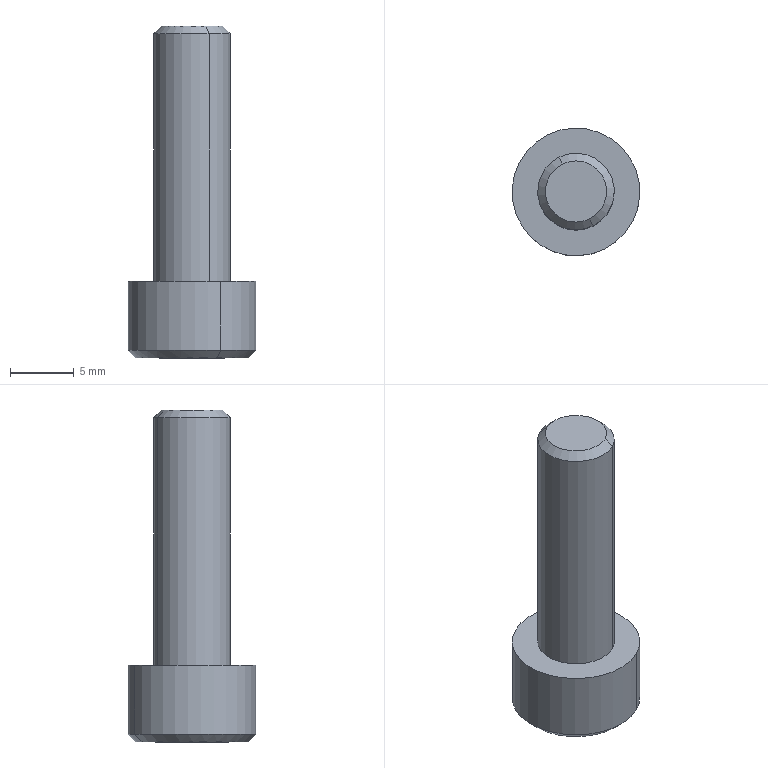Component | SolidWorks | LD101-02-HexagonScrew-M6-2-6 | 1 solid | 25 faces | box 10 x 10 x 26 mm | volume 959 mm3 | plane 15 | cone 6 | cylinder 4 | commonest cylinder face diameters 10 x2 6 x2
STEP:
#1=COLOUR_RGB('',0.7922,0.8196,0.9333);
#2=FILL_AREA_STYLE_COLOUR('',#1);
#3=FILL_AREA_STYLE('',(#2));
#4=SURFACE_STYLE_FILL_AREA(#3);
#5=SURFACE_SIDE_STYLE('',(#4));
#6=SURFACE_STYLE_USAGE(.BOTH.,#5);
#7=PRESENTATION_STYLE_ASSIGNMENT((#6));
#8=CARTESIAN_POINT('',(3.096,-6.841,0.2857));
#9=VERTEX_POINT('',#8);
#10=CARTESIAN_POINT('',(3.18,-7.01,0.2857));
#11=VERTEX_POINT('',#10);
#12=CARTESIAN_POINT('',(3.138,-6.925,0.2857));
#13=DIRECTION('',(0.,0.,1.));
#14=DIRECTION('',(-0.4466,0.8947,0.));
#15=AXIS2_PLACEMENT_3D('',#12,#13,#14);
#16=CIRCLE('',#15,0.09449);
#17=EDGE_CURVE('',#9,#11,#16,.T.);
#18=ORIENTED_EDGE('',*,*,#17,.F.);
#19=CARTESIAN_POINT('',(3.085,-6.819,0.2621));
#20=VERTEX_POINT('',#19);
#21=CARTESIAN_POINT('',(3.096,-6.841,0.2857));
#22=DIRECTION('',(-0.3158,0.6327,-0.7071));
#23=VECTOR('',#22,39.37);
#24=LINE('',#21,#23);
#25=EDGE_CURVE('',#9,#20,#24,.T.);
#26=ORIENTED_EDGE('',*,*,#25,.T.);
#27=CARTESIAN_POINT('',(3.191,-7.031,0.2621));
#28=VERTEX_POINT('',#27);
#29=CARTESIAN_POINT('',(3.138,-6.925,0.2621));
#30=DIRECTION('',(0.,0.,-1.));
#31=DIRECTION('',(-0.4466,0.8947,0.));
#32=AXIS2_PLACEMENT_3D('',#29,#30,#31);
#33=CIRCLE('',#32,0.1181);
#34=EDGE_CURVE('',#28,#20,#33,.T.);
#35=ORIENTED_EDGE('',*,*,#34,.F.);
#36=CARTESIAN_POINT('',(3.18,-7.01,0.2857));
#37=DIRECTION('',(0.3158,-0.6327,-0.7071));
#38=VECTOR('',#37,39.37);
#39=LINE('',#36,#38);
#40=EDGE_CURVE('',#11,#28,#39,.T.);
#41=ORIENTED_EDGE('',*,*,#40,.F.);
#42=EDGE_LOOP('',(#18,#26,#35,#41));
#43=FACE_OUTER_BOUND('',#42,.T.);
#44=CARTESIAN_POINT('',(3.138,-6.925,0.2857));
#45=DIRECTION('',(0.,0.,-1.));
#46=DIRECTION('',(0.4466,-0.8947,0.));
#47=AXIS2_PLACEMENT_3D('',#44,#45,#46);
#48=CONICAL_SURFACE('',#47,0.09449,0.7854);
#49=ADVANCED_FACE('',(#43),#48,.T.);
#50=CARTESIAN_POINT('',(3.05,-6.749,-0.7143));
#51=VERTEX_POINT('',#50);
#52=CARTESIAN_POINT('',(3.226,-7.101,-0.7143));
#53=VERTEX_POINT('',#52);
#54=CARTESIAN_POINT('',(3.138,-6.925,-0.7143));
#55=DIRECTION('',(0.,0.,1.));
#56=DIRECTION('',(-0.4466,0.8947,0.));
#57=AXIS2_PLACEMENT_3D('',#54,#55,#56);
#58=CIRCLE('',#57,0.1969);
#59=EDGE_CURVE('',#51,#53,#58,.T.);
#60=ORIENTED_EDGE('',*,*,#59,.T.);
#61=CARTESIAN_POINT('',(3.226,-7.101,-0.5017));
#62=VERTEX_POINT('',#61);
#63=CARTESIAN_POINT('',(3.226,-7.101,-0.608));
#64=DIRECTION('',(0.,0.,1.));
#65=VECTOR('',#64,39.37);
#66=LINE('',#63,#65);
#67=EDGE_CURVE('',#53,#62,#66,.T.);
#68=ORIENTED_EDGE('',*,*,#67,.T.);
#69=CARTESIAN_POINT('',(3.05,-6.749,-0.5017));
#70=VERTEX_POINT('',#69);
#71=CARTESIAN_POINT('',(3.138,-6.925,-0.5017));
#72=DIRECTION('',(0.,0.,-1.));
#73=DIRECTION('',(-0.4466,0.8947,0.));
#74=AXIS2_PLACEMENT_3D('',#71,#72,#73);
#75=CIRCLE('',#74,0.1969);
#76=EDGE_CURVE('',#62,#70,#75,.T.);
#77=ORIENTED_EDGE('',*,*,#76,.T.);
#78=CARTESIAN_POINT('',(3.05,-6.749,-0.608));
#79=DIRECTION('',(0.,0.,1.));
#80=VECTOR('',#79,39.37);
#81=LINE('',#78,#80);
#82=EDGE_CURVE('',#51,#70,#81,.T.);
#83=ORIENTED_EDGE('',*,*,#82,.F.);
#84=EDGE_LOOP('',(#60,#68,#77,#83));
#85=FACE_OUTER_BOUND('',#84,.T.);
#86=CARTESIAN_POINT('',(3.138,-6.925,-0.608));
#87=DIRECTION('',(0.,0.,1.));
#88=DIRECTION('',(-0.4466,0.8947,0.));
#89=AXIS2_PLACEMENT_3D('',#86,#87,#88);
#90=CYLINDRICAL_SURFACE('',#89,0.1969);
#91=ADVANCED_FACE('',(#85),#90,.T.);
#92=CARTESIAN_POINT('',(3.061,-6.77,-0.7379));
#93=VERTEX_POINT('',#92);
#94=CARTESIAN_POINT('',(3.216,-7.08,-0.7379));
#95=VERTEX_POINT('',#94);
#96=CARTESIAN_POINT('',(3.138,-6.925,-0.7379));
#97=DIRECTION('',(0.,0.,1.));
#98=DIRECTION('',(-0.4466,0.8947,0.));
#99=AXIS2_PLACEMENT_3D('',#96,#97,#98);
#100=CIRCLE('',#99,0.1732);
#101=EDGE_CURVE('',#93,#95,#100,.T.);
#102=ORIENTED_EDGE('',*,*,#101,.T.);
#103=CARTESIAN_POINT('',(3.226,-7.101,-0.7143));
#104=DIRECTION('',(0.3158,-0.6327,0.7071));
#105=VECTOR('',#104,39.37);
#106=LINE('',#103,#105);
#107=EDGE_CURVE('',#95,#53,#106,.T.);
#108=ORIENTED_EDGE('',*,*,#107,.T.);
#109=ORIENTED_EDGE('',*,*,#59,.F.);
#110=CARTESIAN_POINT('',(3.05,-6.749,-0.7143));
#111=DIRECTION('',(-0.3158,0.6327,0.7071));
#112=VECTOR('',#111,39.37);
#113=LINE('',#110,#112);
#114=EDGE_CURVE('',#93,#51,#113,.T.);
#115=ORIENTED_EDGE('',*,*,#114,.F.);
#116=EDGE_LOOP('',(#102,#108,#109,#115));
#117=FACE_OUTER_BOUND('',#116,.T.);
#118=CARTESIAN_POINT('',(3.138,-6.925,-0.7143));
#119=DIRECTION('',(0.,0.,1.));
#120=DIRECTION('',(-0.4466,0.8947,0.));
#121=AXIS2_PLACEMENT_3D('',#118,#119,#120);
#122=CONICAL_SURFACE('',#121,0.1969,0.7854);
#123=ADVANCED_FACE('',(#117),#122,.T.);
#124=CARTESIAN_POINT('',(3.191,-7.031,-0.5017));
#125=VERTEX_POINT('',#124);
#126=CARTESIAN_POINT('',(3.085,-6.819,-0.5017));
#127=VERTEX_POINT('',#126);
#128=CARTESIAN_POINT('',(3.138,-6.925,-0.5017));
#129=DIRECTION('',(0.,0.,-1.));
#130=DIRECTION('',(-0.4466,0.8947,0.));
#131=AXIS2_PLACEMENT_3D('',#128,#129,#130);
#132=CIRCLE('',#131,0.1181);
#133=EDGE_CURVE('',#125,#127,#132,.T.);
#134=ORIENTED_EDGE('',*,*,#133,.F.);
#135=CARTESIAN_POINT('',(3.191,-7.031,-0.3563));
#136=DIRECTION('',(0.,0.,1.));
#137=VECTOR('',#136,39.37);
#138=LINE('',#135,#137);
#139=EDGE_CURVE('',#125,#28,#138,.T.);
#140=ORIENTED_EDGE('',*,*,#139,.T.);
#141=ORIENTED_EDGE('',*,*,#34,.T.);
#142=CARTESIAN_POINT('',(3.085,-6.819,-0.3563));
#143=DIRECTION('',(0.,0.,1.));
#144=VECTOR('',#143,39.37);
#145=LINE('',#142,#144);
#146=EDGE_CURVE('',#127,#20,#145,.T.);
#147=ORIENTED_EDGE('',*,*,#146,.F.);
#148=EDGE_LOOP('',(#134,#140,#141,#147));
#149=FACE_OUTER_BOUND('',#148,.T.);
#150=CARTESIAN_POINT('',(3.138,-6.925,-0.3563));
#151=DIRECTION('',(0.,0.,1.));
#152=DIRECTION('',(-0.4466,0.8947,0.));
#153=AXIS2_PLACEMENT_3D('',#150,#151,#152);
#154=CYLINDRICAL_SURFACE('',#153,0.1181);
#155=ADVANCED_FACE('',(#149),#154,.T.);
#156=CARTESIAN_POINT('',(3.138,-6.925,-0.5934));
#157=VERTEX_POINT('',#156);
#158=CARTESIAN_POINT('',(3.182,-7.013,-0.6198));
#159=VERTEX_POINT('',#158);
#160=CARTESIAN_POINT('',(3.182,-7.013,-0.6198));
#161=DIRECTION('',(0.4314,-0.8642,-0.2588));
#162=VECTOR('',#161,39.37);
#163=LINE('',#160,#162);
#164=EDGE_CURVE('',#157,#159,#163,.T.);
#165=ORIENTED_EDGE('',*,*,#164,.F.);
#166=CARTESIAN_POINT('',(3.094,-6.837,-0.6198));
#167=VERTEX_POINT('',#166);
#168=CARTESIAN_POINT('',(3.094,-6.837,-0.6198));
#169=DIRECTION('',(-0.4314,0.8642,-0.2588));
#170=VECTOR('',#169,39.37);
#171=LINE('',#168,#170);
#172=EDGE_CURVE('',#157,#167,#171,.T.);
#173=ORIENTED_EDGE('',*,*,#172,.T.);
#174=CARTESIAN_POINT('',(3.192,-6.843,-0.6198));
#175=VERTEX_POINT('',#174);
#176=CARTESIAN_POINT('',(3.138,-6.925,-0.6198));
#177=DIRECTION('',(0.,-0.,1.));
#178=DIRECTION('',(0.4466,-0.8947,0.));
#179=AXIS2_PLACEMENT_3D('',#176,#177,#178);
#180=CIRCLE('',#179,0.09843);
#181=EDGE_CURVE('',#175,#167,#180,.T.);
#182=ORIENTED_EDGE('',*,*,#181,.F.);
#183=CARTESIAN_POINT('',(3.236,-6.931,-0.6198));
#184=VERTEX_POINT('',#183);
#185=CARTESIAN_POINT('',(3.138,-6.925,-0.6198));
#186=DIRECTION('',(0.,-0.,1.));
#187=DIRECTION('',(0.4466,-0.8947,0.));
#188=AXIS2_PLACEMENT_3D('',#185,#186,#187);
#189=CIRCLE('',#188,0.09843);
#190=EDGE_CURVE('',#184,#175,#189,.T.);
#191=ORIENTED_EDGE('',*,*,#190,.F.);
#192=CARTESIAN_POINT('',(3.138,-6.925,-0.6198));
#193=DIRECTION('',(-0.,0.,-1.));
#194=DIRECTION('',(0.4466,-0.8947,0.));
#195=AXIS2_PLACEMENT_3D('',#192,#193,#194);
#196=CIRCLE('',#195,0.09843);
#197=EDGE_CURVE('',#184,#159,#196,.T.);
#198=ORIENTED_EDGE('',*,*,#197,.T.);
#199=EDGE_LOOP('',(#165,#173,#182,#191,#198));
#200=FACE_OUTER_BOUND('',#199,.T.);
#201=CARTESIAN_POINT('',(3.138,-6.925,-0.6198));
#202=DIRECTION('',(-0.,0.,-1.));
#203=DIRECTION('',(0.4466,-0.8947,0.));
#204=AXIS2_PLACEMENT_3D('',#201,#202,#203);
#205=CONICAL_SURFACE('',#204,0.09843,1.309);
#206=ADVANCED_FACE('',(#200),#205,.F.);
#207=ORIENTED_EDGE('',*,*,#67,.F.);
#208=CARTESIAN_POINT('',(3.138,-6.925,-0.7143));
#209=DIRECTION('',(0.,0.,1.));
#210=DIRECTION('',(-0.4466,0.8947,0.));
#211=AXIS2_PLACEMENT_3D('',#208,#209,#210);
#212=CIRCLE('',#211,0.1969);
#213=EDGE_CURVE('',#53,#51,#212,.T.);
#214=ORIENTED_EDGE('',*,*,#213,.T.);
#215=ORIENTED_EDGE('',*,*,#82,.T.);
#216=CARTESIAN_POINT('',(3.138,-6.925,-0.5017));
#217=DIRECTION('',(0.,0.,-1.));
#218=DIRECTION('',(-0.4466,0.8947,0.));
#219=AXIS2_PLACEMENT_3D('',#216,#217,#218);
#220=CIRCLE('',#219,0.1969);
#221=EDGE_CURVE('',#70,#62,#220,.T.);
#222=ORIENTED_EDGE('',*,*,#221,.T.);
#223=EDGE_LOOP('',(#207,#214,#215,#222));
#224=FACE_OUTER_BOUND('',#223,.T.);
#225=CARTESIAN_POINT('',(3.138,-6.925,-0.608));
#226=DIRECTION('',(0.,0.,1.));
#227=DIRECTION('',(-0.4466,0.8947,0.));
#228=AXIS2_PLACEMENT_3D('',#225,#226,#227);
#229=CYLINDRICAL_SURFACE('',#228,0.1969);
#230=ADVANCED_FACE('',(#224),#229,.T.);
#231=ORIENTED_EDGE('',*,*,#107,.F.);
#232=CARTESIAN_POINT('',(3.138,-6.925,-0.7379));
#233=DIRECTION('',(0.,0.,1.));
#234=DIRECTION('',(-0.4466,0.8947,0.));
#235=AXIS2_PLACEMENT_3D('',#232,#233,#234);
#236=CIRCLE('',#235,0.1732);
#237=EDGE_CURVE('',#95,#93,#236,.T.);
#238=ORIENTED_EDGE('',*,*,#237,.T.);
#239=ORIENTED_EDGE('',*,*,#114,.T.);
#240=ORIENTED_EDGE('',*,*,#213,.F.);
#241=EDGE_LOOP('',(#231,#238,#239,#240));
#242=FACE_OUTER_BOUND('',#241,.T.);
#243=CARTESIAN_POINT('',(3.138,-6.925,-0.7143));
#244=DIRECTION('',(0.,0.,1.));
#245=DIRECTION('',(-0.4466,0.8947,0.));
#246=AXIS2_PLACEMENT_3D('',#243,#244,#245);
#247=CONICAL_SURFACE('',#246,0.1969,0.7854);
#248=ADVANCED_FACE('',(#242),#247,.T.);
#249=CARTESIAN_POINT('',(3.138,-6.925,-0.5017));
#250=DIRECTION('',(0.,0.,-1.));
#251=DIRECTION('',(-0.4466,0.8947,0.));
#252=AXIS2_PLACEMENT_3D('',#249,#250,#251);
#253=CIRCLE('',#252,0.1181);
#254=EDGE_CURVE('',#127,#125,#253,.T.);
#255=ORIENTED_EDGE('',*,*,#254,.T.);
#256=ORIENTED_EDGE('',*,*,#133,.T.);
#257=EDGE_LOOP('',(#255,#256));
#258=FACE_BOUND('',#257,.T.);
#259=ORIENTED_EDGE('',*,*,#221,.F.);
#260=ORIENTED_EDGE('',*,*,#76,.F.);
#261=EDGE_LOOP('',(#259,#260));
#262=FACE_OUTER_BOUND('',#261,.T.);
#263=CARTESIAN_POINT('',(2.997,-6.995,-0.5017));
#264=DIRECTION('',(0.,0.,1.));
#265=DIRECTION('',(-0.4466,0.8947,0.));
#266=AXIS2_PLACEMENT_3D('',#263,#264,#265);
#267=PLANE('',#266);
#268=ADVANCED_FACE('',(#258,#262),#267,.T.);
#269=ORIENTED_EDGE('',*,*,#101,.F.);
#270=ORIENTED_EDGE('',*,*,#237,.F.);
#271=EDGE_LOOP('',(#269,#270));
#272=FACE_OUTER_BOUND('',#271,.T.);
#273=CARTESIAN_POINT('',(3.043,-6.862,-0.7379));
#274=VERTEX_POINT('',#273);
#275=CARTESIAN_POINT('',(3.037,-6.976,-0.7379));
#276=VERTEX_POINT('',#275);
#277=CARTESIAN_POINT('',(3.043,-6.862,-0.7379));
#278=DIRECTION('',(-0.06055,-0.9982,0.));
#279=VECTOR('',#278,39.37);
#280=LINE('',#277,#279);
#281=EDGE_CURVE('',#274,#276,#280,.T.);
#282=ORIENTED_EDGE('',*,*,#281,.T.);
#283=CARTESIAN_POINT('',(3.131,-7.039,-0.7379));
#284=VERTEX_POINT('',#283);
#285=CARTESIAN_POINT('',(3.037,-6.976,-0.7379));
#286=DIRECTION('',(0.8342,-0.5515,0.));
#287=VECTOR('',#286,39.37);
#288=LINE('',#285,#287);
#289=EDGE_CURVE('',#276,#284,#288,.T.);
#290=ORIENTED_EDGE('',*,*,#289,.T.);
#291=CARTESIAN_POINT('',(3.233,-6.988,-0.7379));
#292=VERTEX_POINT('',#291);
#293=CARTESIAN_POINT('',(3.105,-7.052,-0.7379));
#294=DIRECTION('',(0.8947,0.4466,0.));
#295=VECTOR('',#294,39.37);
#296=LINE('',#293,#295);
#297=EDGE_CURVE('',#284,#292,#296,.T.);
#298=ORIENTED_EDGE('',*,*,#297,.T.);
#299=CARTESIAN_POINT('',(3.24,-6.874,-0.7379));
#300=VERTEX_POINT('',#299);
#301=CARTESIAN_POINT('',(3.233,-6.988,-0.7379));
#302=DIRECTION('',(0.06055,0.9982,0.));
#303=VECTOR('',#302,39.37);
#304=LINE('',#301,#303);
#305=EDGE_CURVE('',#292,#300,#304,.T.);
#306=ORIENTED_EDGE('',*,*,#305,.T.);
#307=CARTESIAN_POINT('',(3.145,-6.812,-0.7379));
#308=VERTEX_POINT('',#307);
#309=CARTESIAN_POINT('',(3.24,-6.874,-0.7379));
#310=DIRECTION('',(-0.8342,0.5515,0.));
#311=VECTOR('',#310,39.37);
#312=LINE('',#309,#311);
#313=EDGE_CURVE('',#300,#308,#312,.T.);
#314=ORIENTED_EDGE('',*,*,#313,.T.);
#315=CARTESIAN_POINT('',(3.017,-6.876,-0.7379));
#316=DIRECTION('',(-0.8947,-0.4466,0.));
#317=VECTOR('',#316,39.37);
#318=LINE('',#315,#317);
#319=EDGE_CURVE('',#308,#274,#318,.T.);
#320=ORIENTED_EDGE('',*,*,#319,.T.);
#321=EDGE_LOOP('',(#282,#290,#298,#306,#314,#320));
#322=FACE_BOUND('',#321,.T.);
#323=CARTESIAN_POINT('',(3.061,-6.964,-0.7379));
#324=DIRECTION('',(0.,0.,-1.));
#325=DIRECTION('',(0.4466,-0.8947,0.));
#326=AXIS2_PLACEMENT_3D('',#323,#324,#325);
#327=PLANE('',#326);
#328=ADVANCED_FACE('',(#272,#322),#327,.T.);
#329=ORIENTED_EDGE('',*,*,#139,.F.);
#330=ORIENTED_EDGE('',*,*,#254,.F.);
#331=ORIENTED_EDGE('',*,*,#146,.T.);
#332=CARTESIAN_POINT('',(3.138,-6.925,0.2621));
#333=DIRECTION('',(0.,0.,-1.));
#334=DIRECTION('',(-0.4466,0.8947,0.));
#335=AXIS2_PLACEMENT_3D('',#332,#333,#334);
#336=CIRCLE('',#335,0.1181);
#337=EDGE_CURVE('',#20,#28,#336,.T.);
#338=ORIENTED_EDGE('',*,*,#337,.T.);
#339=EDGE_LOOP('',(#329,#330,#331,#338));
#340=FACE_OUTER_BOUND('',#339,.T.);
#341=CARTESIAN_POINT('',(3.138,-6.925,-0.3563));
#342=DIRECTION('',(0.,0.,1.));
#343=DIRECTION('',(-0.4466,0.8947,0.));
#344=AXIS2_PLACEMENT_3D('',#341,#342,#343);
#345=CYLINDRICAL_SURFACE('',#344,0.1181);
#346=ADVANCED_FACE('',(#340),#345,.T.);
#347=CARTESIAN_POINT('',(3.037,-6.976,-0.6198));
#348=VERTEX_POINT('',#347);
#349=CARTESIAN_POINT('',(3.037,-6.976,-0.7379));
#350=DIRECTION('',(0.,0.,-1.));
#351=VECTOR('',#350,39.37);
#352=LINE('',#349,#351);
#353=EDGE_CURVE('',#348,#276,#352,.T.);
#354=ORIENTED_EDGE('',*,*,#353,.F.);
#355=CARTESIAN_POINT('',(3.084,-7.007,-0.6198));
#356=VERTEX_POINT('',#355);
#357=CARTESIAN_POINT('',(3.131,-7.039,-0.6198));
#358=DIRECTION('',(-0.8342,0.5515,0.));
#359=VECTOR('',#358,39.37);
#360=LINE('',#357,#359);
#361=EDGE_CURVE('',#356,#348,#360,.T.);
#362=ORIENTED_EDGE('',*,*,#361,.F.);
#363=CARTESIAN_POINT('',(3.131,-7.039,-0.6198));
#364=VERTEX_POINT('',#363);
#365=CARTESIAN_POINT('',(3.084,-7.007,-0.6198));
#366=DIRECTION('',(0.8342,-0.5515,0.));
#367=VECTOR('',#366,39.37);
#368=LINE('',#365,#367);
#369=EDGE_CURVE('',#356,#364,#368,.T.);
#370=ORIENTED_EDGE('',*,*,#369,.T.);
#371=CARTESIAN_POINT('',(3.131,-7.039,-0.7379));
#372=DIRECTION('',(0.,0.,1.));
#373=VECTOR('',#372,39.37);
#374=LINE('',#371,#373);
#375=EDGE_CURVE('',#284,#364,#374,.T.);
#376=ORIENTED_EDGE('',*,*,#375,.F.);
#377=ORIENTED_EDGE('',*,*,#289,.F.);
#378=EDGE_LOOP('',(#354,#362,#370,#376,#377));
#379=FACE_OUTER_BOUND('',#378,.T.);
#380=CARTESIAN_POINT('',(3.131,-7.039,-0.7379));
#381=DIRECTION('',(-0.5515,-0.8342,0.));
#382=DIRECTION('',(0.8342,-0.5515,0.));
#383=AXIS2_PLACEMENT_3D('',#380,#381,#382);
#384=PLANE('',#383);
#385=ADVANCED_FACE('',(#379),#384,.F.);
#386=CARTESIAN_POINT('',(3.043,-6.862,-0.6198));
#387=VERTEX_POINT('',#386);
#388=CARTESIAN_POINT('',(3.043,-6.862,-0.7379));
#389=DIRECTION('',(0.,0.,-1.));
#390=VECTOR('',#389,39.37);
#391=LINE('',#388,#390);
#392=EDGE_CURVE('',#387,#274,#391,.T.);
#393=ORIENTED_EDGE('',*,*,#392,.F.);
#394=CARTESIAN_POINT('',(3.04,-6.919,-0.6198));
#395=VERTEX_POINT('',#394);
#396=CARTESIAN_POINT('',(3.043,-6.862,-0.6198));
#397=DIRECTION('',(-0.06055,-0.9982,0.));
#398=VECTOR('',#397,39.37);
#399=LINE('',#396,#398);
#400=EDGE_CURVE('',#387,#395,#399,.T.);
#401=ORIENTED_EDGE('',*,*,#400,.T.);
#402=CARTESIAN_POINT('',(3.037,-6.976,-0.6198));
#403=DIRECTION('',(0.06055,0.9982,0.));
#404=VECTOR('',#403,39.37);
#405=LINE('',#402,#404);
#406=EDGE_CURVE('',#348,#395,#405,.T.);
#407=ORIENTED_EDGE('',*,*,#406,.F.);
#408=ORIENTED_EDGE('',*,*,#353,.T.);
#409=ORIENTED_EDGE('',*,*,#281,.F.);
#410=EDGE_LOOP('',(#393,#401,#407,#408,#409));
#411=FACE_OUTER_BOUND('',#410,.T.);
#412=CARTESIAN_POINT('',(3.037,-6.976,-0.7379));
#413=DIRECTION('',(-0.9982,0.06055,0.));
#414=DIRECTION('',(-0.06055,-0.9982,0.));
#415=AXIS2_PLACEMENT_3D('',#412,#413,#414);
#416=PLANE('',#415);
#417=ADVANCED_FACE('',(#411),#416,.F.);
#418=CARTESIAN_POINT('',(3.145,-6.812,-0.6198));
#419=VERTEX_POINT('',#418);
#420=CARTESIAN_POINT('',(3.145,-6.812,-0.7379));
#421=DIRECTION('',(0.,0.,-1.));
#422=VECTOR('',#421,39.37);
#423=LINE('',#420,#422);
#424=EDGE_CURVE('',#419,#308,#423,.T.);
#425=ORIENTED_EDGE('',*,*,#424,.F.);
#426=CARTESIAN_POINT('',(3.094,-6.837,-0.6198));
#427=DIRECTION('',(-0.8947,-0.4466,0.));
#428=VECTOR('',#427,39.37);
#429=LINE('',#426,#428);
#430=EDGE_CURVE('',#419,#167,#429,.T.);
#431=ORIENTED_EDGE('',*,*,#430,.T.);
#432=CARTESIAN_POINT('',(3.094,-6.837,-0.6198));
#433=DIRECTION('',(-0.8947,-0.4466,0.));
#434=VECTOR('',#433,39.37);
#435=LINE('',#432,#434);
#436=EDGE_CURVE('',#167,#387,#435,.T.);
#437=ORIENTED_EDGE('',*,*,#436,.T.);
#438=ORIENTED_EDGE('',*,*,#392,.T.);
#439=ORIENTED_EDGE('',*,*,#319,.F.);
#440=EDGE_LOOP('',(#425,#431,#437,#438,#439));
#441=FACE_OUTER_BOUND('',#440,.T.);
#442=CARTESIAN_POINT('',(3.043,-6.862,-0.7379));
#443=DIRECTION('',(-0.4466,0.8947,0.));
#444=DIRECTION('',(0.,0.,-1.));
#445=AXIS2_PLACEMENT_3D('',#442,#443,#444);
#446=PLANE('',#445);
#447=ADVANCED_FACE('',(#441),#446,.F.);
#448=CARTESIAN_POINT('',(3.24,-6.874,-0.6198));
#449=VERTEX_POINT('',#448);
#450=CARTESIAN_POINT('',(3.24,-6.874,-0.7379));
#451=DIRECTION('',(0.,0.,-1.));
#452=VECTOR('',#451,39.37);
#453=LINE('',#450,#452);
#454=EDGE_CURVE('',#449,#300,#453,.T.);
#455=ORIENTED_EDGE('',*,*,#454,.F.);
#456=CARTESIAN_POINT('',(3.145,-6.812,-0.6198));
#457=DIRECTION('',(0.8342,-0.5515,0.));
#458=VECTOR('',#457,39.37);
#459=LINE('',#456,#458);
#460=EDGE_CURVE('',#175,#449,#459,.T.);
#461=ORIENTED_EDGE('',*,*,#460,.F.);
#462=CARTESIAN_POINT('',(3.192,-6.843,-0.6198));
#463=DIRECTION('',(-0.8342,0.5515,0.));
#464=VECTOR('',#463,39.37);
#465=LINE('',#462,#464);
#466=EDGE_CURVE('',#175,#419,#465,.T.);
#467=ORIENTED_EDGE('',*,*,#466,.T.);
#468=ORIENTED_EDGE('',*,*,#424,.T.);
#469=ORIENTED_EDGE('',*,*,#313,.F.);
#470=EDGE_LOOP('',(#455,#461,#467,#468,#469));
#471=FACE_OUTER_BOUND('',#470,.T.);
#472=CARTESIAN_POINT('',(3.145,-6.812,-0.7379));
#473=DIRECTION('',(0.5515,0.8342,0.));
#474=DIRECTION('',(-0.8342,0.5515,0.));
#475=AXIS2_PLACEMENT_3D('',#472,#473,#474);
#476=PLANE('',#475);
#477=ADVANCED_FACE('',(#471),#476,.F.);
#478=CARTESIAN_POINT('',(3.233,-6.988,-0.6198));
#479=VERTEX_POINT('',#478);
#480=CARTESIAN_POINT('',(3.233,-6.988,-0.7379));
#481=DIRECTION('',(0.,0.,-1.));
#482=VECTOR('',#481,39.37);
#483=LINE('',#480,#482);
#484=EDGE_CURVE('',#479,#292,#483,.T.);
#485=ORIENTED_EDGE('',*,*,#484,.F.);
#486=CARTESIAN_POINT('',(3.24,-6.874,-0.6198));
#487=DIRECTION('',(-0.06055,-0.9982,0.));
#488=VECTOR('',#487,39.37);
#489=LINE('',#486,#488);
#490=EDGE_CURVE('',#184,#479,#489,.T.);
#491=ORIENTED_EDGE('',*,*,#490,.F.);
#492=CARTESIAN_POINT('',(3.24,-6.874,-0.6198));
#493=DIRECTION('',(-0.06055,-0.9982,0.));
#494=VECTOR('',#493,39.37);
#495=LINE('',#492,#494);
#496=EDGE_CURVE('',#449,#184,#495,.T.);
#497=ORIENTED_EDGE('',*,*,#496,.F.);
#498=ORIENTED_EDGE('',*,*,#454,.T.);
#499=ORIENTED_EDGE('',*,*,#305,.F.);
#500=EDGE_LOOP('',(#485,#491,#497,#498,#499));
#501=FACE_OUTER_BOUND('',#500,.T.);
#502=CARTESIAN_POINT('',(3.24,-6.874,-0.7379));
#503=DIRECTION('',(0.9982,-0.06055,0.));
#504=DIRECTION('',(0.06055,0.9982,0.));
#505=AXIS2_PLACEMENT_3D('',#502,#503,#504);
#506=PLANE('',#505);
#507=ADVANCED_FACE('',(#501),#506,.F.);
#508=ORIENTED_EDGE('',*,*,#375,.T.);
#509=CARTESIAN_POINT('',(3.182,-7.013,-0.6198));
#510=DIRECTION('',(0.8947,0.4466,0.));
#511=VECTOR('',#510,39.37);
#512=LINE('',#509,#511);
#513=EDGE_CURVE('',#364,#159,#512,.T.);
#514=ORIENTED_EDGE('',*,*,#513,.T.);
#515=CARTESIAN_POINT('',(3.233,-6.988,-0.6198));
#516=DIRECTION('',(-0.8947,-0.4466,0.));
#517=VECTOR('',#516,39.37);
#518=LINE('',#515,#517);
#519=EDGE_CURVE('',#479,#159,#518,.T.);
#520=ORIENTED_EDGE('',*,*,#519,.F.);
#521=ORIENTED_EDGE('',*,*,#484,.T.);
#522=ORIENTED_EDGE('',*,*,#297,.F.);
#523=EDGE_LOOP('',(#508,#514,#520,#521,#522));
#524=FACE_OUTER_BOUND('',#523,.T.);
#525=CARTESIAN_POINT('',(3.233,-6.988,-0.7379));
#526=DIRECTION('',(0.4466,-0.8947,0.));
#527=DIRECTION('',(0.,0.,1.));
#528=AXIS2_PLACEMENT_3D('',#525,#526,#527);
#529=PLANE('',#528);
#530=ADVANCED_FACE('',(#524),#529,.F.);
#531=ORIENTED_EDGE('',*,*,#361,.T.);
#532=ORIENTED_EDGE('',*,*,#406,.T.);
#533=CARTESIAN_POINT('',(3.138,-6.925,-0.6198));
#534=DIRECTION('',(0.,-0.,1.));
#535=DIRECTION('',(0.4466,-0.8947,0.));
#536=AXIS2_PLACEMENT_3D('',#533,#534,#535);
#537=CIRCLE('',#536,0.09843);
#538=EDGE_CURVE('',#395,#356,#537,.T.);
#539=ORIENTED_EDGE('',*,*,#538,.T.);
#540=EDGE_LOOP('',(#531,#532,#539));
#541=FACE_OUTER_BOUND('',#540,.T.);
#542=CARTESIAN_POINT('',(3.138,-6.925,-0.6198));
#543=DIRECTION('',(0.,0.,1.));
#544=DIRECTION('',(-0.4466,0.8947,0.));
#545=AXIS2_PLACEMENT_3D('',#542,#543,#544);
#546=PLANE('',#545);
#547=ADVANCED_FACE('',(#541),#546,.F.);
#548=ORIENTED_EDGE('',*,*,#460,.T.);
#549=ORIENTED_EDGE('',*,*,#496,.T.);
#550=ORIENTED_EDGE('',*,*,#190,.T.);
#551=EDGE_LOOP('',(#548,#549,#550));
#552=FACE_OUTER_BOUND('',#551,.T.);
#553=CARTESIAN_POINT('',(3.138,-6.925,-0.6198));
#554=DIRECTION('',(0.,0.,1.));
#555=DIRECTION('',(-0.4466,0.8947,0.));
#556=AXIS2_PLACEMENT_3D('',#553,#554,#555);
#557=PLANE('',#556);
#558=ADVANCED_FACE('',(#552),#557,.F.);
#559=ORIENTED_EDGE('',*,*,#490,.T.);
#560=ORIENTED_EDGE('',*,*,#519,.T.);
#561=ORIENTED_EDGE('',*,*,#197,.F.);
#562=EDGE_LOOP('',(#559,#560,#561));
#563=FACE_OUTER_BOUND('',#562,.T.);
#564=CARTESIAN_POINT('',(3.138,-6.925,-0.6198));
#565=DIRECTION('',(0.,0.,1.));
#566=DIRECTION('',(-0.4466,0.8947,0.));
#567=AXIS2_PLACEMENT_3D('',#564,#565,#566);
#568=PLANE('',#567);
#569=ADVANCED_FACE('',(#563),#568,.F.);
#570=ORIENTED_EDGE('',*,*,#172,.F.);
#571=ORIENTED_EDGE('',*,*,#164,.T.);
#572=CARTESIAN_POINT('',(3.138,-6.925,-0.6198));
#573=DIRECTION('',(0.,-0.,1.));
#574=DIRECTION('',(0.4466,-0.8947,0.));
#575=AXIS2_PLACEMENT_3D('',#572,#573,#574);
#576=CIRCLE('',#575,0.09843);
#577=EDGE_CURVE('',#356,#159,#576,.T.);
#578=ORIENTED_EDGE('',*,*,#577,.F.);
#579=ORIENTED_EDGE('',*,*,#538,.F.);
#580=CARTESIAN_POINT('',(3.138,-6.925,-0.6198));
#581=DIRECTION('',(0.,-0.,1.));
#582=DIRECTION('',(0.4466,-0.8947,0.));
#583=AXIS2_PLACEMENT_3D('',#580,#581,#582);
#584=CIRCLE('',#583,0.09843);
#585=EDGE_CURVE('',#167,#395,#584,.T.);
#586=ORIENTED_EDGE('',*,*,#585,.F.);
#587=EDGE_LOOP('',(#570,#571,#578,#579,#586));
#588=FACE_OUTER_BOUND('',#587,.T.);
#589=CARTESIAN_POINT('',(3.138,-6.925,-0.6198));
#590=DIRECTION('',(-0.,0.,-1.));
#591=DIRECTION('',(0.4466,-0.8947,0.));
#592=AXIS2_PLACEMENT_3D('',#589,#590,#591);
#593=CONICAL_SURFACE('',#592,0.09843,1.309);
#594=ADVANCED_FACE('',(#588),#593,.F.);
#595=ORIENTED_EDGE('',*,*,#513,.F.);
#596=ORIENTED_EDGE('',*,*,#369,.F.);
#597=ORIENTED_EDGE('',*,*,#577,.T.);
#598=EDGE_LOOP('',(#595,#596,#597));
#599=FACE_OUTER_BOUND('',#598,.T.);
#600=CARTESIAN_POINT('',(3.138,-6.925,-0.6198));
#601=DIRECTION('',(0.,0.,1.));
#602=DIRECTION('',(-0.4466,0.8947,0.));
#603=AXIS2_PLACEMENT_3D('',#600,#601,#602);
#604=PLANE('',#603);
#605=ADVANCED_FACE('',(#599),#604,.F.);
#606=ORIENTED_EDGE('',*,*,#400,.F.);
#607=ORIENTED_EDGE('',*,*,#436,.F.);
#608=ORIENTED_EDGE('',*,*,#585,.T.);
#609=EDGE_LOOP('',(#606,#607,#608));
#610=FACE_OUTER_BOUND('',#609,.T.);
#611=CARTESIAN_POINT('',(3.138,-6.925,-0.6198));
#612=DIRECTION('',(0.,0.,1.));
#613=DIRECTION('',(-0.4466,0.8947,0.));
#614=AXIS2_PLACEMENT_3D('',#611,#612,#613);
#615=PLANE('',#614);
#616=ADVANCED_FACE('',(#610),#615,.F.);
#617=ORIENTED_EDGE('',*,*,#430,.F.);
#618=ORIENTED_EDGE('',*,*,#466,.F.);
#619=ORIENTED_EDGE('',*,*,#181,.T.);
#620=EDGE_LOOP('',(#617,#618,#619));
#621=FACE_OUTER_BOUND('',#620,.T.);
#622=CARTESIAN_POINT('',(3.138,-6.925,-0.6198));
#623=DIRECTION('',(0.,0.,1.));
#624=DIRECTION('',(-0.4466,0.8947,0.));
#625=AXIS2_PLACEMENT_3D('',#622,#623,#624);
#626=PLANE('',#625);
#627=ADVANCED_FACE('',(#621),#626,.F.);
#628=CARTESIAN_POINT('',(3.138,-6.925,0.2857));
#629=DIRECTION('',(0.,0.,1.));
#630=DIRECTION('',(-0.4466,0.8947,0.));
#631=AXIS2_PLACEMENT_3D('',#628,#629,#630);
#632=CIRCLE('',#631,0.09449);
#633=EDGE_CURVE('',#11,#9,#632,.T.);
#634=ORIENTED_EDGE('',*,*,#633,.T.);
#635=ORIENTED_EDGE('',*,*,#17,.T.);
#636=EDGE_LOOP('',(#634,#635));
#637=FACE_OUTER_BOUND('',#636,.T.);
#638=CARTESIAN_POINT('',(3.138,-6.925,0.2857));
#639=DIRECTION('',(0.,0.,1.));
#640=DIRECTION('',(-0.4466,0.8947,0.));
#641=AXIS2_PLACEMENT_3D('',#638,#639,#640);
#642=PLANE('',#641);
#643=ADVANCED_FACE('',(#637),#642,.T.);
#644=ORIENTED_EDGE('',*,*,#25,.F.);
#645=ORIENTED_EDGE('',*,*,#633,.F.);
#646=ORIENTED_EDGE('',*,*,#40,.T.);
#647=ORIENTED_EDGE('',*,*,#337,.F.);
#648=EDGE_LOOP('',(#644,#645,#646,#647));
#649=FACE_OUTER_BOUND('',#648,.T.);
#650=CARTESIAN_POINT('',(3.138,-6.925,0.2857));
#651=DIRECTION('',(0.,0.,-1.));
#652=DIRECTION('',(0.4466,-0.8947,0.));
#653=AXIS2_PLACEMENT_3D('',#650,#651,#652);
#654=CONICAL_SURFACE('',#653,0.09449,0.7854);
#655=ADVANCED_FACE('',(#649),#654,.T.);
#656=CLOSED_SHELL('',(#49,#91,#123,#155,#206,#230,#248,#268,#328,#346,#385,#417,#447,#477,#507,#530,#547,#558,#569,#594,#605,#616,#627,#643,#655));
#657=MANIFOLD_SOLID_BREP('',#656);
#658=STYLED_ITEM('',(#7),#657);
#659=(LENGTH_UNIT()NAMED_UNIT(*)SI_UNIT($,.METRE.));
#660=LENGTH_MEASURE_WITH_UNIT(LENGTH_MEASURE(0.0254),#659);
#661=DIMENSIONAL_EXPONENTS(1.,0.,0.,0.,0.,0.,0.);
#662=(CONVERSION_BASED_UNIT('',#660)LENGTH_UNIT()NAMED_UNIT(#661));
#663=UNCERTAINTY_MEASURE_WITH_UNIT(LENGTH_MEASURE(0.00001),#662,'','');
#664=(NAMED_UNIT(*)PLANE_ANGLE_UNIT()SI_UNIT($,.RADIAN.));
#665=(NAMED_UNIT(*)SI_UNIT($,.STERADIAN.)SOLID_ANGLE_UNIT());
#666=(GEOMETRIC_REPRESENTATION_CONTEXT(3)GLOBAL_UNCERTAINTY_ASSIGNED_CONTEXT((#663))GLOBAL_UNIT_ASSIGNED_CONTEXT((#662,#664,#665))REPRESENTATION_CONTEXT('',''));
#667=MECHANICAL_DESIGN_GEOMETRIC_PRESENTATION_REPRESENTATION('',(#658),#666);
#668=CARTESIAN_POINT('',(0.,0.,0.));
#669=DIRECTION('',(0.,0.,1.));
#670=DIRECTION('',(1.,0.,0.));
#671=AXIS2_PLACEMENT_3D('',#668,#669,#670);
#672=(LENGTH_UNIT()NAMED_UNIT(*)SI_UNIT($,.METRE.));
#673=LENGTH_MEASURE_WITH_UNIT(LENGTH_MEASURE(0.0254),#672);
#674=DIMENSIONAL_EXPONENTS(1.,0.,0.,0.,0.,0.,0.);
#675=(CONVERSION_BASED_UNIT('',#673)LENGTH_UNIT()NAMED_UNIT(#674));
#676=UNCERTAINTY_MEASURE_WITH_UNIT(LENGTH_MEASURE(0.00001),#675,'','');
#677=(NAMED_UNIT(*)PLANE_ANGLE_UNIT()SI_UNIT($,.RADIAN.));
#678=(NAMED_UNIT(*)SI_UNIT($,.STERADIAN.)SOLID_ANGLE_UNIT());
#679=(GEOMETRIC_REPRESENTATION_CONTEXT(3)GLOBAL_UNCERTAINTY_ASSIGNED_CONTEXT((#676))GLOBAL_UNIT_ASSIGNED_CONTEXT((#675,#677,#678))REPRESENTATION_CONTEXT('',''));
#680=ADVANCED_BREP_SHAPE_REPRESENTATION('',(#657,#671),#679);
#681=PRESENTATION_LAYER_ASSIGNMENT('','',(#658));